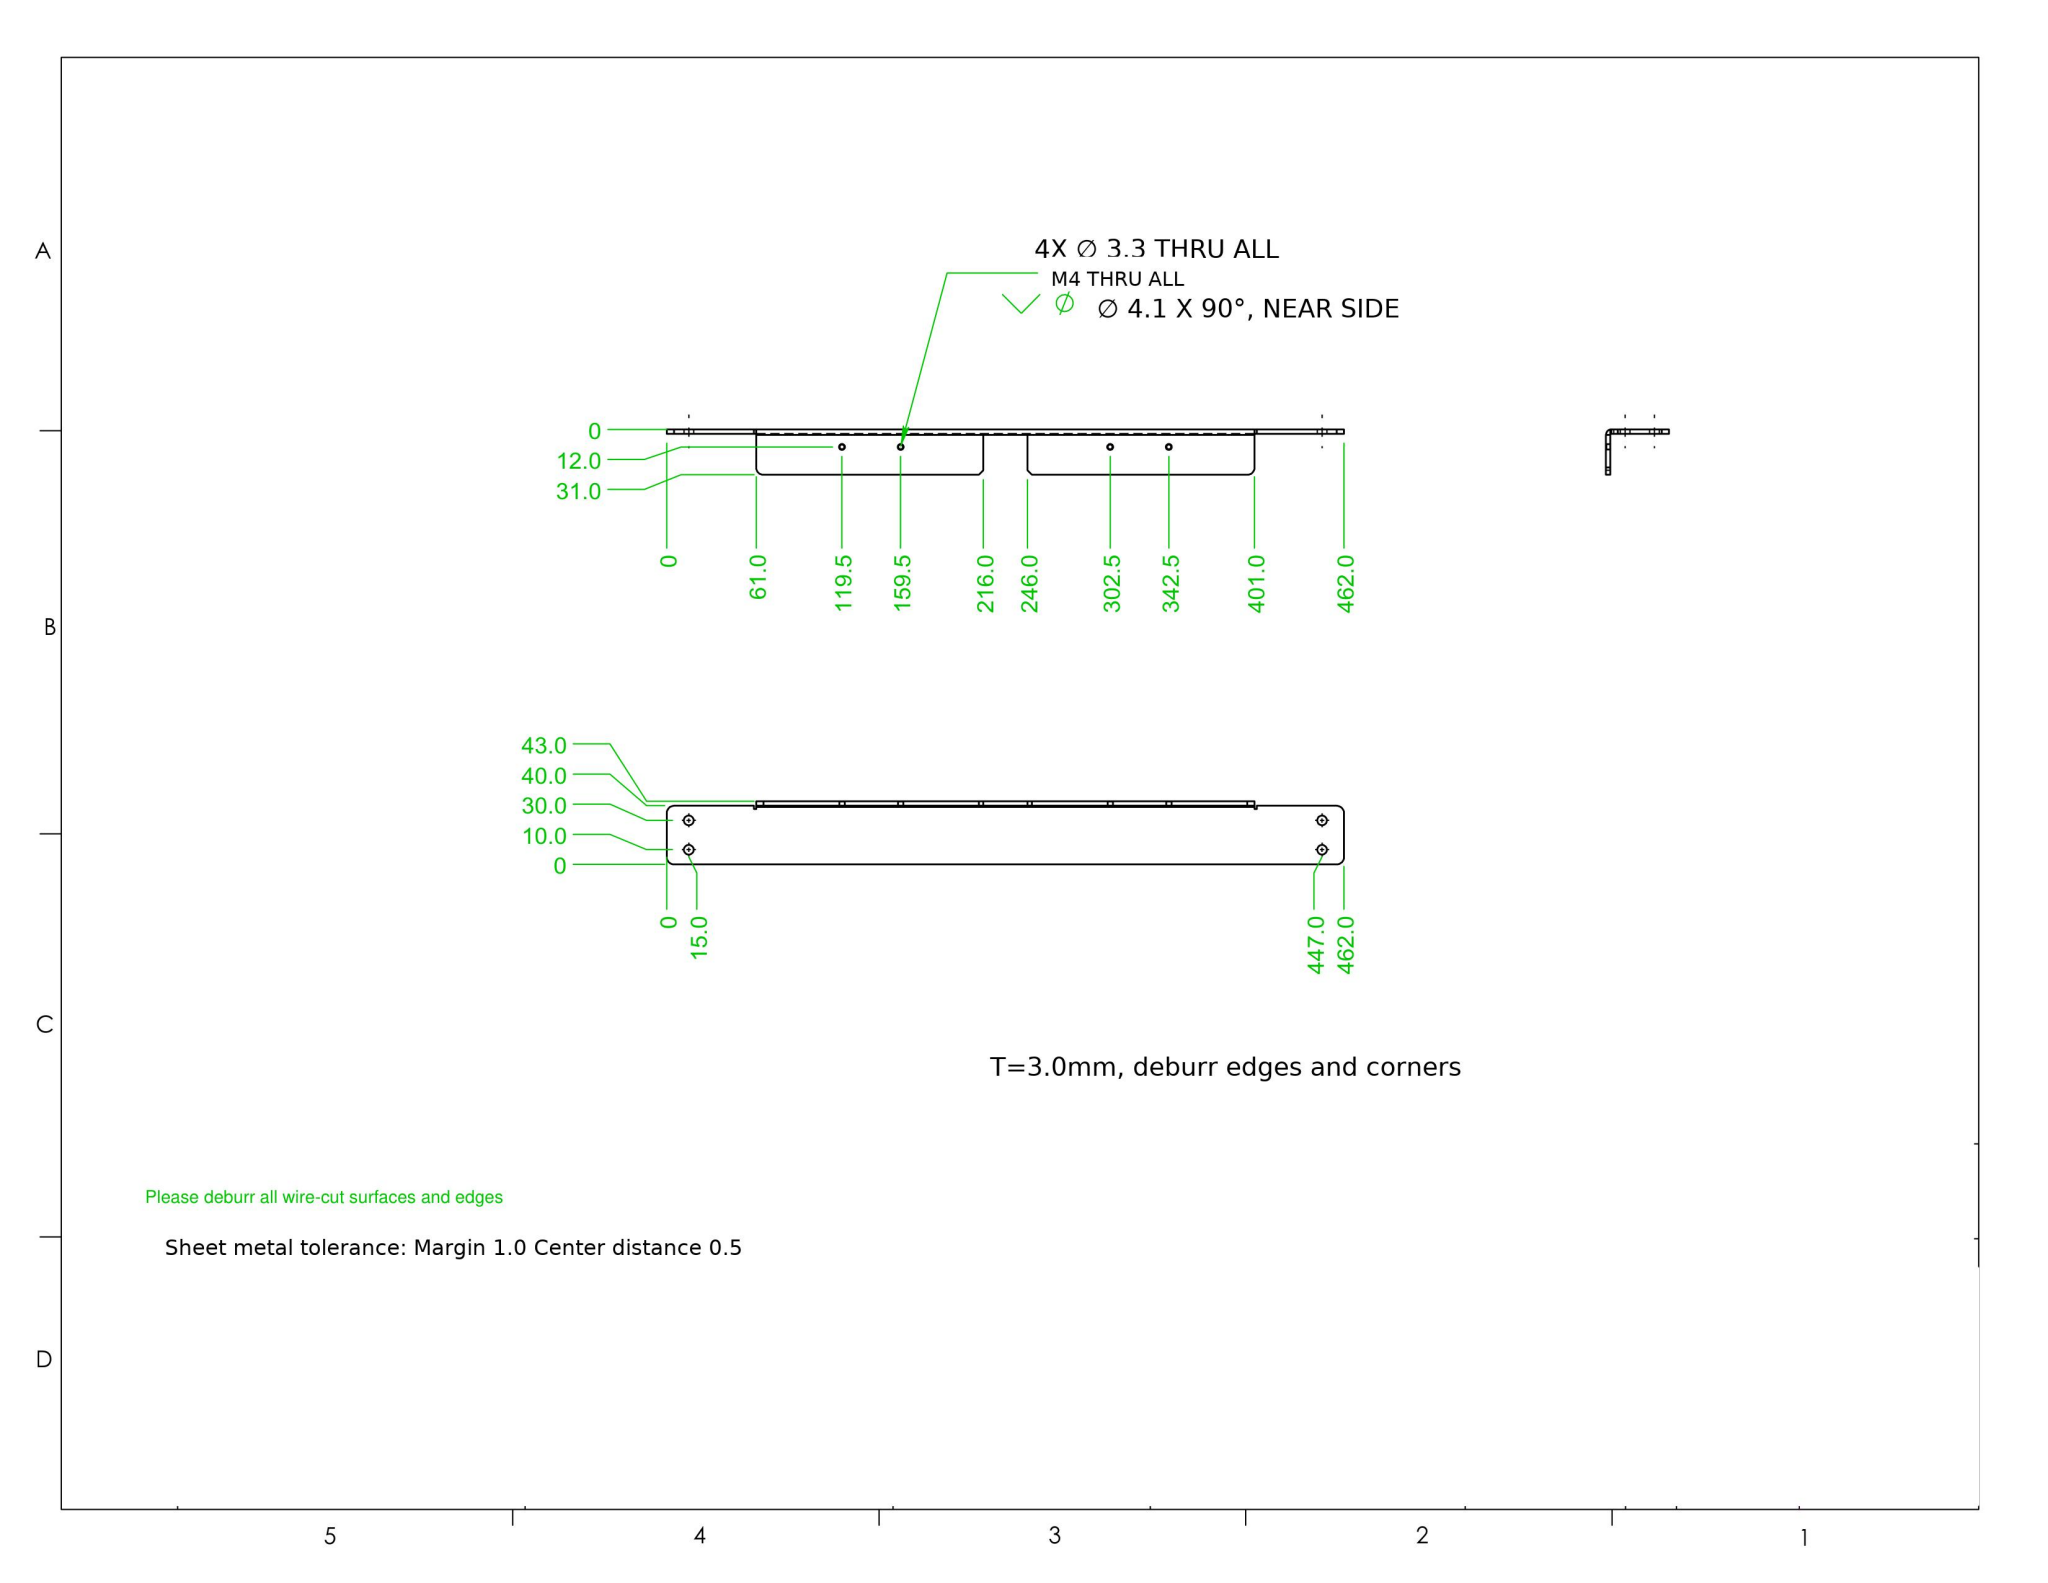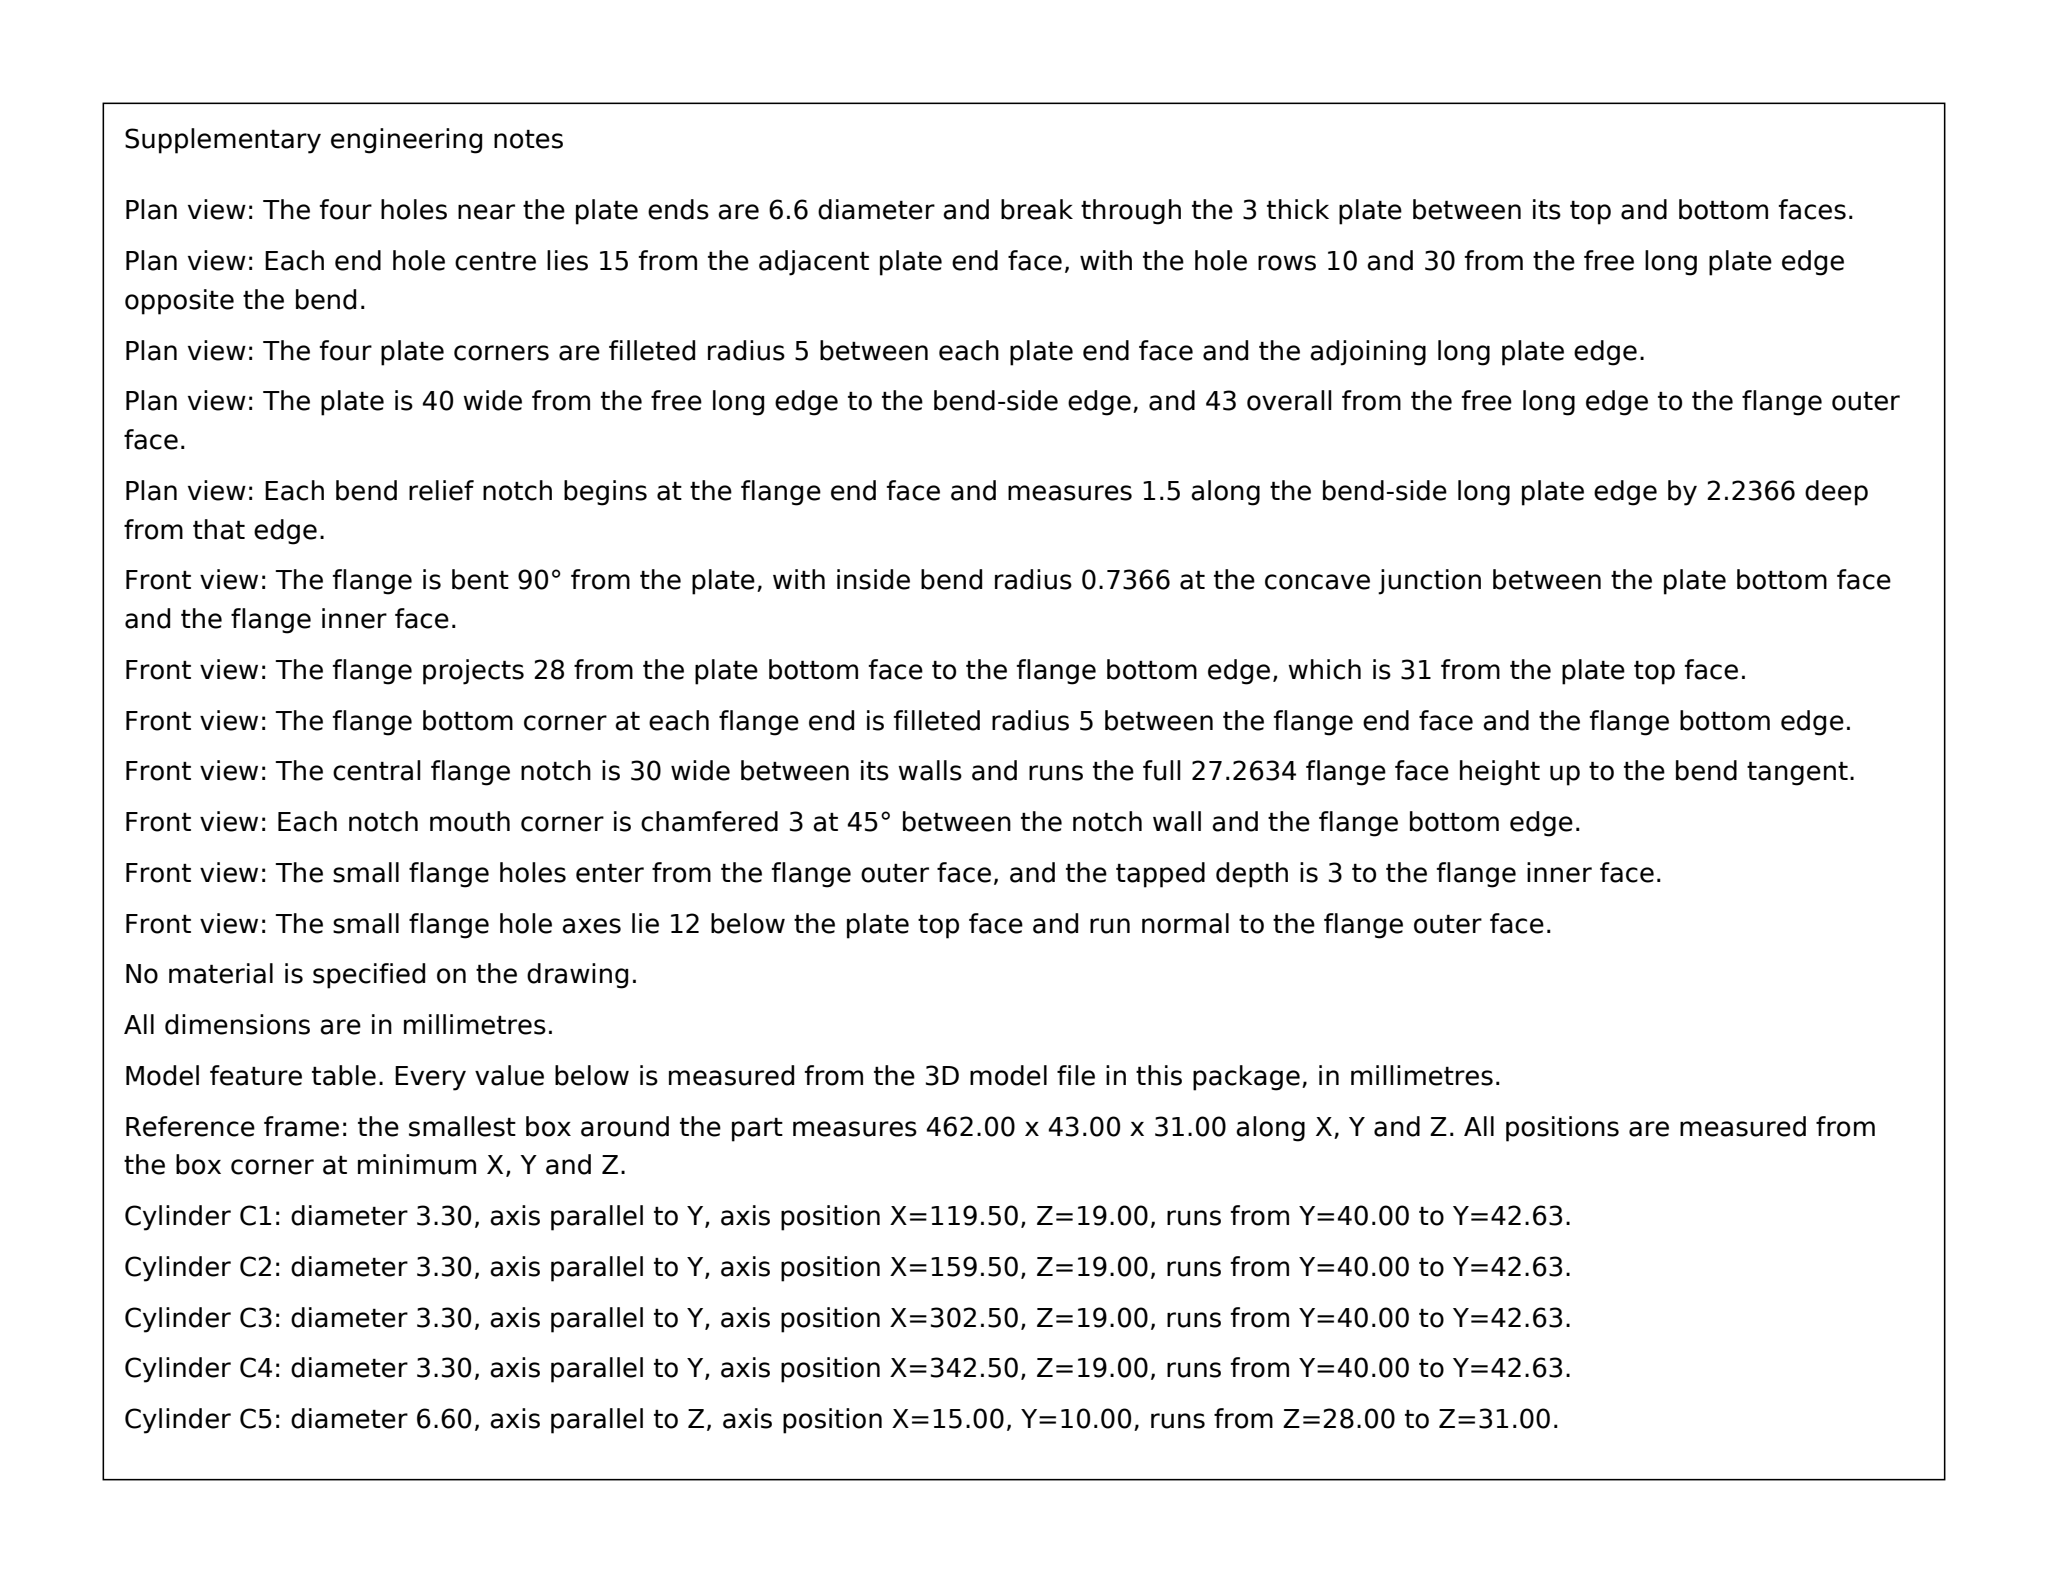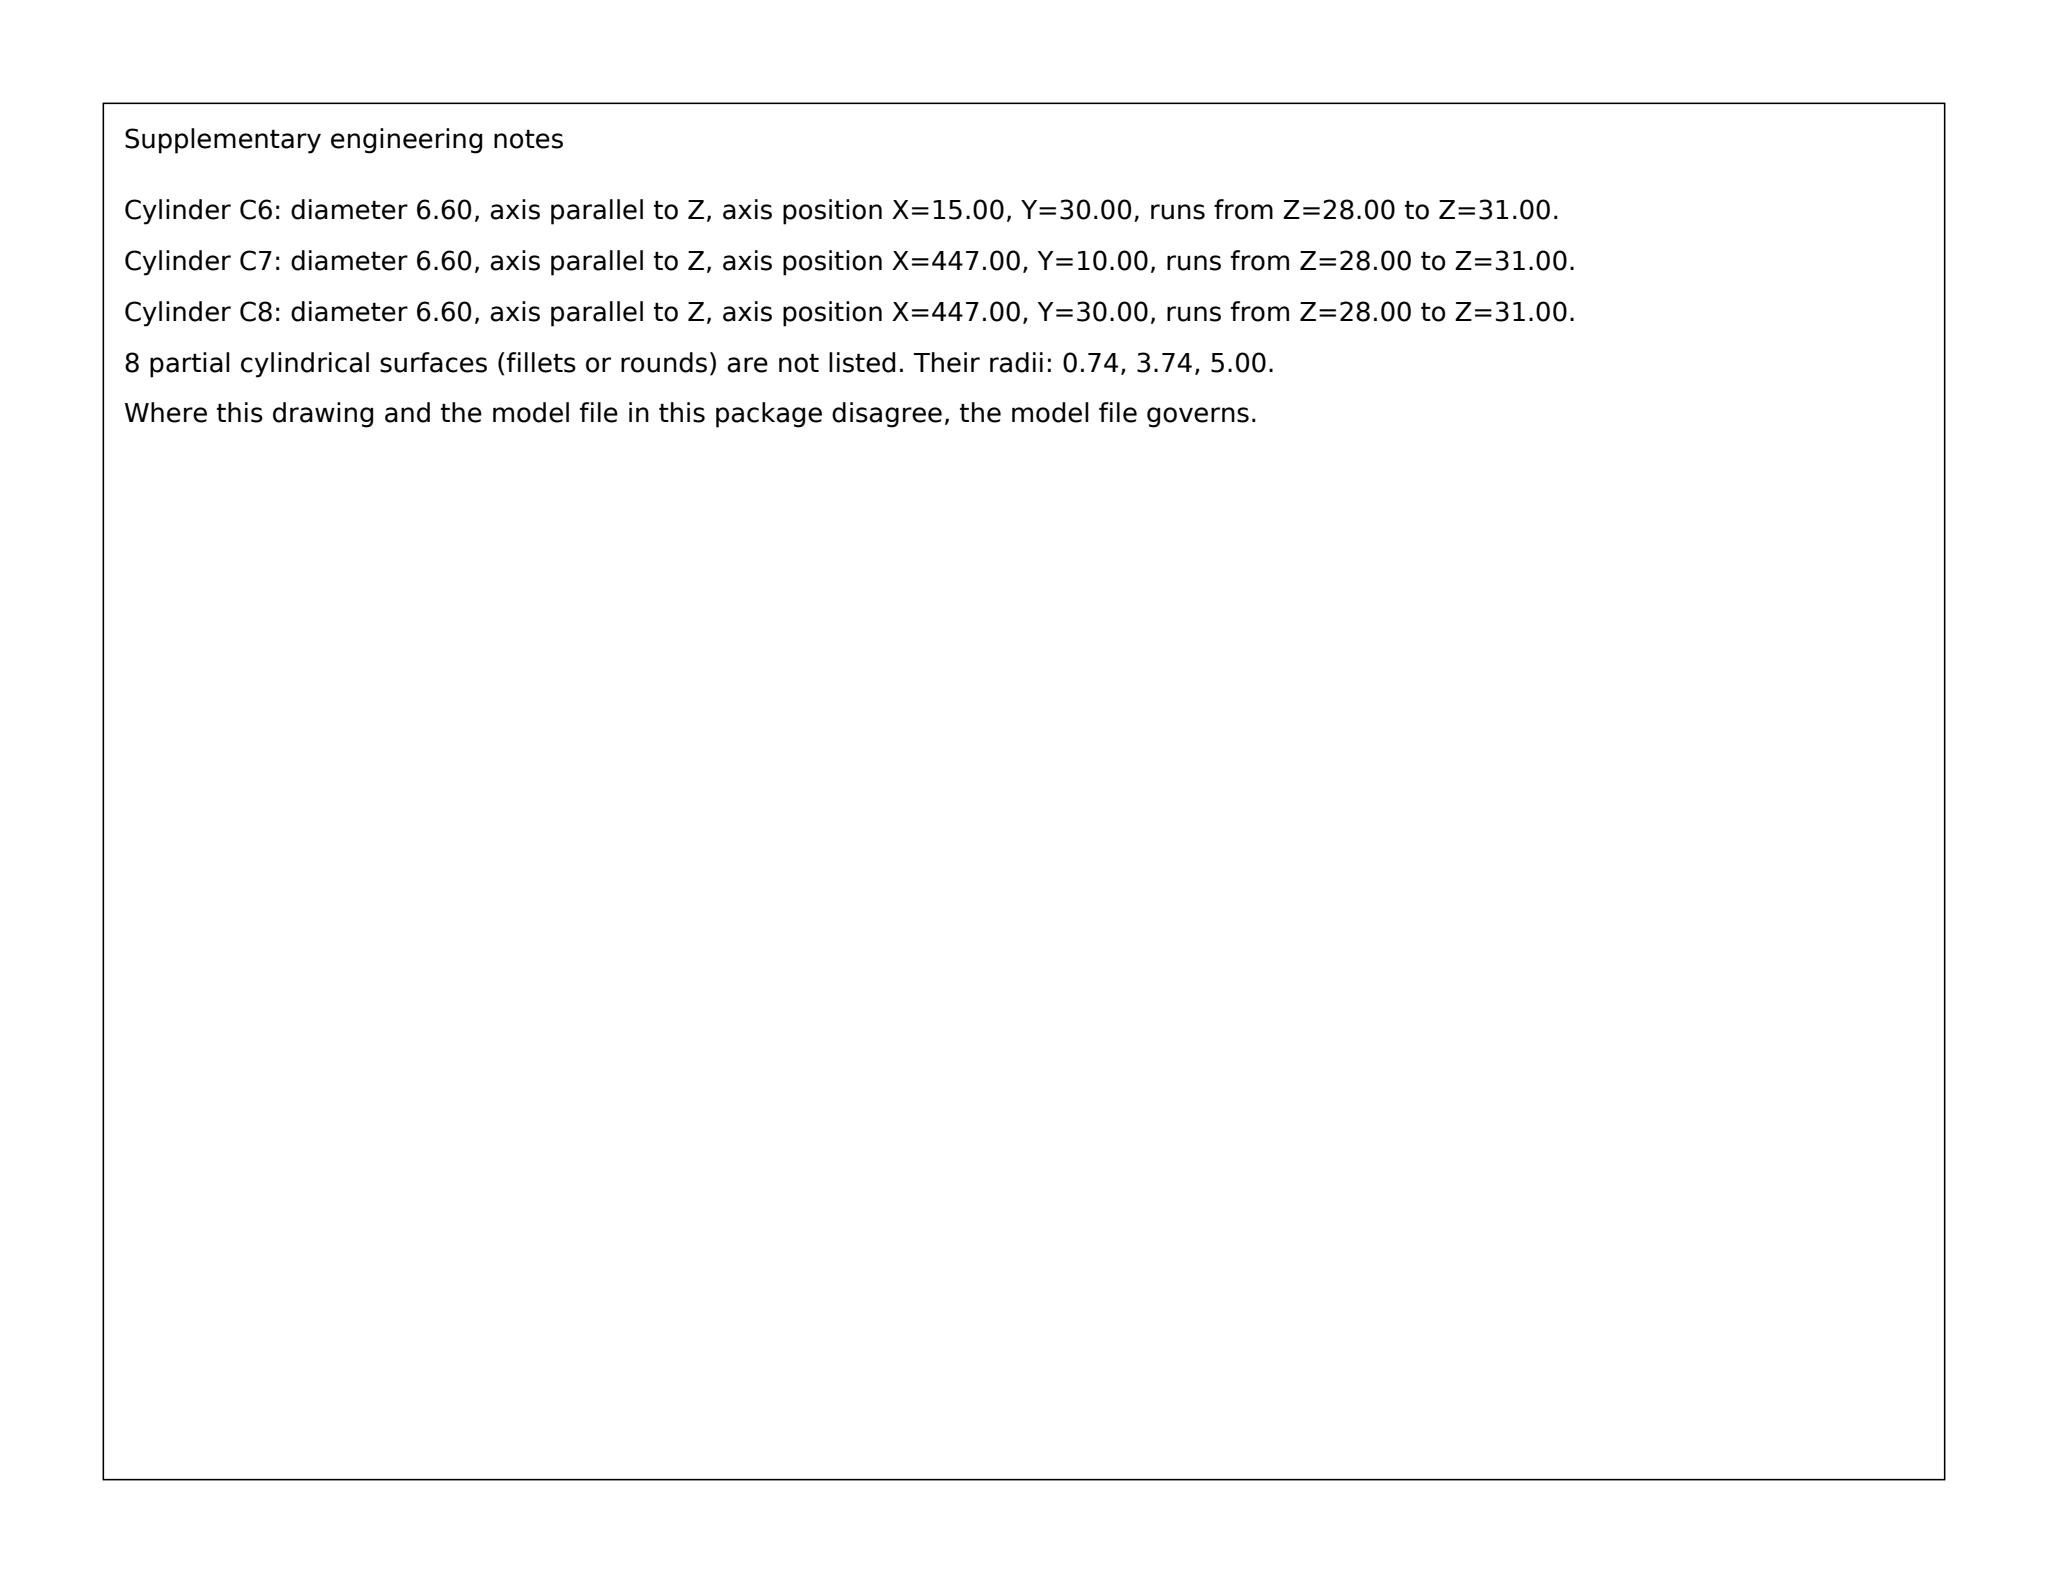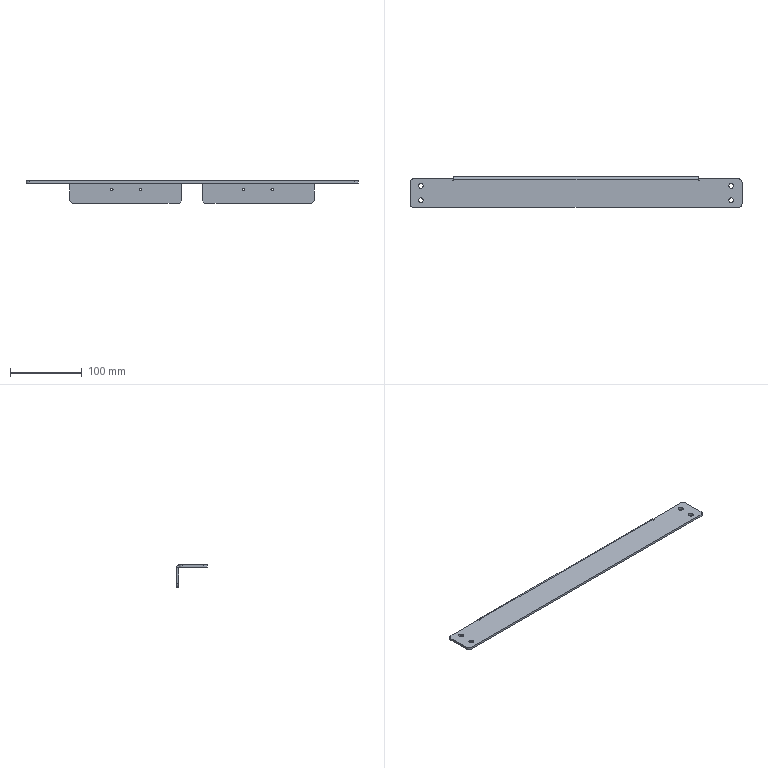Part | SolidWorks | mm | 1 solid | 60 faces | box 462 x 43 x 31 mm | volume 82967 mm3 | plane 28 | cylinder 24 | cone 8 | commonest cylinder face diameters 3.3 x8 6.6 x8 10 x6 7.473 x1 1.473 x1
Drawing notes:
4X Ø6.6 THRU, END PLATES AT X15/447, Y10/30 | from the solid: cylinders dia 6.6 axis z at (15,10),(15,30),(447,10),(447,30), length 3.0
ALL CORNER RADII R5 TYP (END PLATES & X61/401) | from the solid: dia 10.0 cyls at z-corners (5,5),(5,35),(457,5),(457,35) and y-axis at (66,5),(396,5)
FORMED EDGE: INSIDE R0.74, OUTSIDE R3.74, T=3.0 | from the solid: x-axis cylinders dia 1.473 and 7.473 at (y39.26, z27.26), len 340
REAR LIP: LAND 3 (Z28 TO 31), END 2.24 INSIDE Y40 FACE | from the solid: planes z=28, z=31, y=37.76, y=40
2X 1.5 STEP: X59.5 TO 61.0 & X401.0 TO 402.5 | from the solid: x planes at 59.5, 61.0, 401.0, 402.5